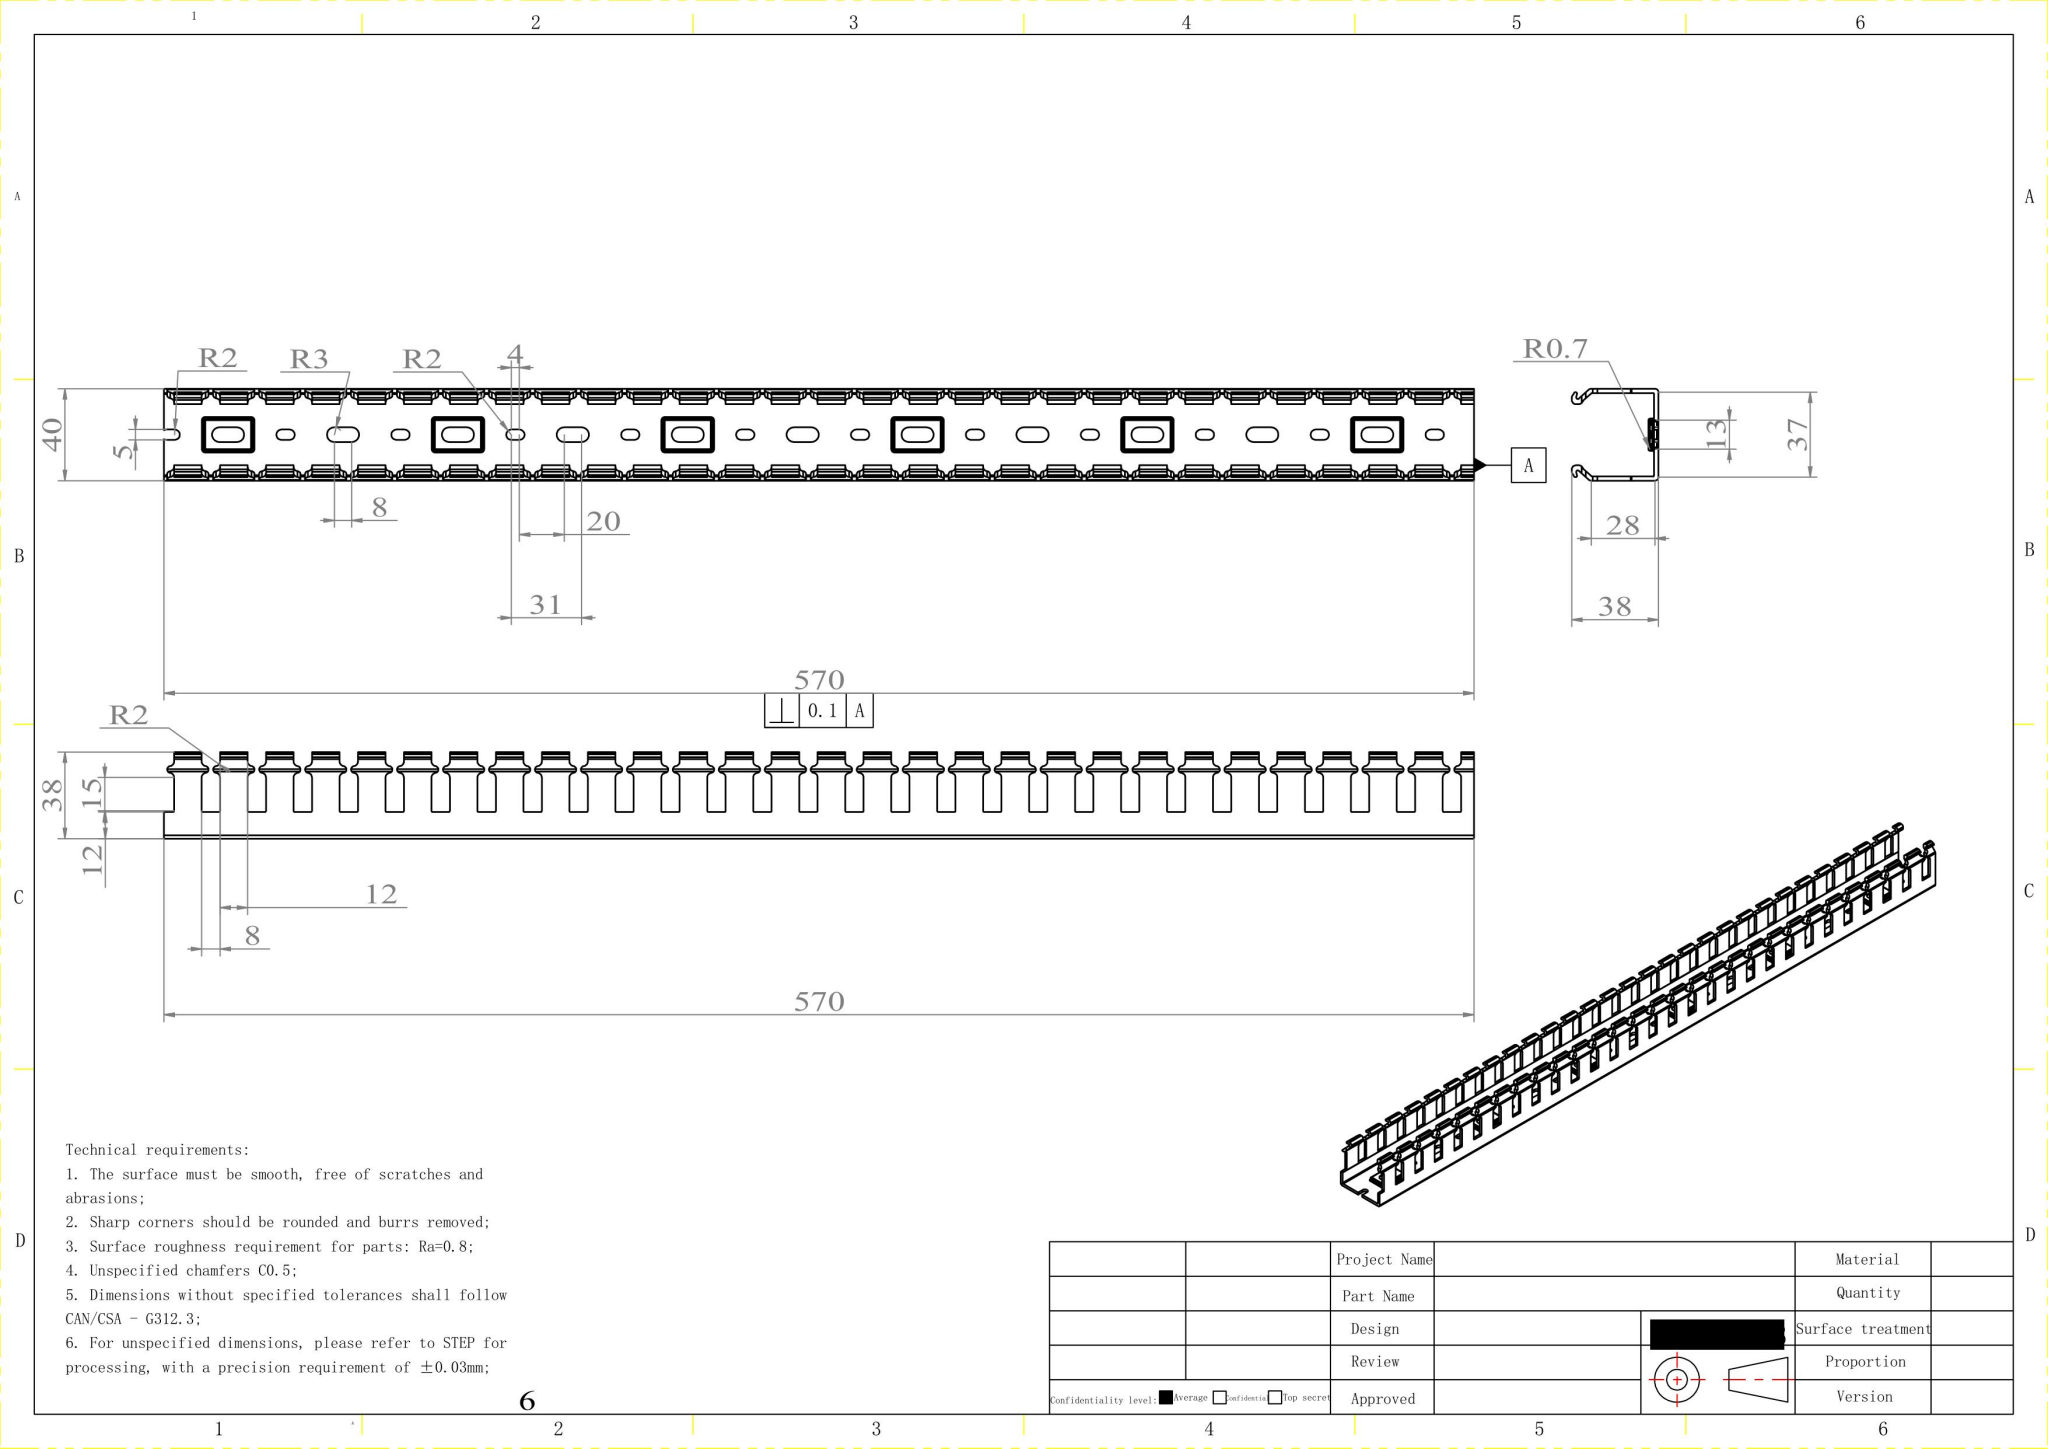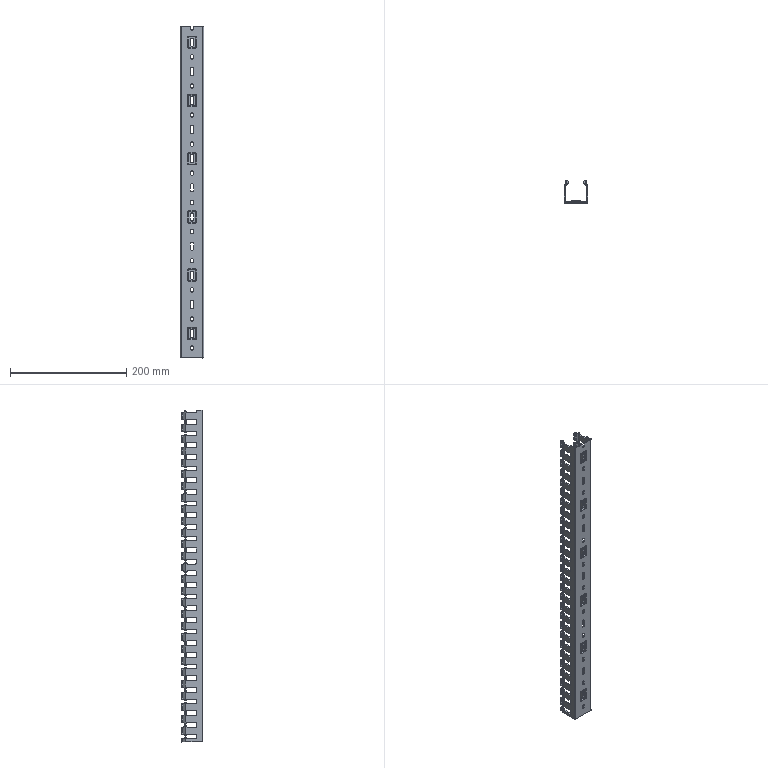Part | SolidWorks | mm | 1 solid | 2191 faces | box 40 x 37.7 x 570 mm | volume 103680 mm3 | cylinder 1234 | plane 813 | sphere 96 | torus 48 | commonest cylinder face diameters 4 x228 1 x178 3 x174 3.6 x174 1.4 x173 1.464 x144 10 x58 6 x58